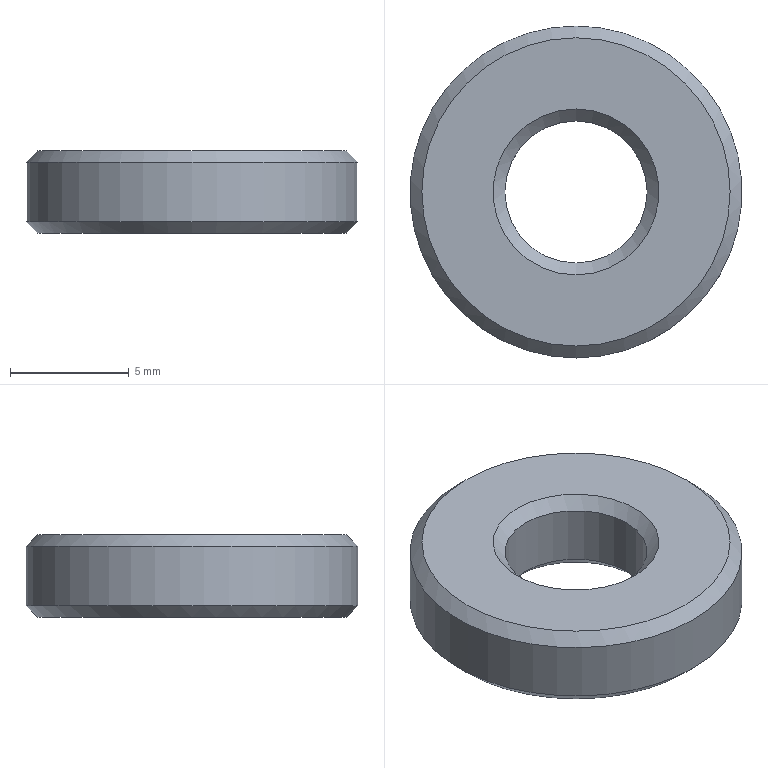Component | NX | STOPPER | 1 solid | 8 faces | box 14 x 14 x 3.5 mm | volume 424 mm3 | cone 4 | cylinder 2 | plane 2 | commonest cylinder face diameters 14 x1 6 x1
STEP:
#1=CARTESIAN_POINT('',(0.,0.,0.));
#2=DIRECTION('',(0.,0.,1.));
#3=DIRECTION('',(1.,0.,0.));
#4=AXIS2_PLACEMENT_3D('',#1,#2,#3);
#5=CARTESIAN_POINT('',(-8.293,7.,-172.611));
#6=VERTEX_POINT('',#5);
#7=CARTESIAN_POINT('',(-8.293,0.,-172.611));
#8=DIRECTION('',(0.,0.,-1.));
#9=DIRECTION('',(0.,1.,0.));
#10=AXIS2_PLACEMENT_3D('',#7,#8,#9);
#11=CIRCLE('',#10,7.);
#12=CARTESIAN_POINT('',(-8.293,0.,-175.611));
#13=DIRECTION('',(0.,0.,1.));
#14=DIRECTION('',(0.,1.,0.));
#15=AXIS2_PLACEMENT_3D('',#12,#13,#14);
#16=CYLINDRICAL_SURFACE('',#15,7.);
#17=CARTESIAN_POINT('',(6.283,3.));
#18=DIRECTION('',(-1.,0.));
#19=VECTOR('',#18,1.);
#20=LINE('',#17,#19);
#21=(GEOMETRIC_REPRESENTATION_CONTEXT(2)PARAMETRIC_REPRESENTATION_CONTEXT()REPRESENTATION_CONTEXT('',''));
#22=DEFINITIONAL_REPRESENTATION('',(#20),#21);
#23=PCURVE('',#16,#22);
#24=CARTESIAN_POINT('',(-8.293,0.,-172.111));
#25=DIRECTION('',(0.,0.,-1.));
#26=DIRECTION('',(0.,-1.,0.));
#27=AXIS2_PLACEMENT_3D('',#24,#25,#26);
#28=CONICAL_SURFACE('',#27,6.5,0.7854);
#29=CARTESIAN_POINT('',(3.142,0.5));
#30=DIRECTION('',(1.,0.));
#31=VECTOR('',#30,1.);
#32=LINE('',#29,#31);
#33=(GEOMETRIC_REPRESENTATION_CONTEXT(2)PARAMETRIC_REPRESENTATION_CONTEXT()REPRESENTATION_CONTEXT('',''));
#34=DEFINITIONAL_REPRESENTATION('',(#32),#33);
#35=PCURVE('',#28,#34);
#36=SURFACE_CURVE('',#11,(#23,#35),.PCURVE_S1.);
#37=EDGE_CURVE('',#6,#6,#36,.T.);
#38=ORIENTED_EDGE('',*,*,#37,.T.);
#39=CARTESIAN_POINT('',(-8.293,7.,-175.111));
#40=VERTEX_POINT('',#39);
#41=CARTESIAN_POINT('',(-8.293,7.,-175.111));
#42=CARTESIAN_POINT('',(-8.293,7.,-172.611));
#43=B_SPLINE_CURVE_WITH_KNOTS('',1,(#41,#42),.UNSPECIFIED.,.F.,.F.,(2,2),(0.5,3.),.PIECEWISE_BEZIER_KNOTS.);
#44=CARTESIAN_POINT('',(0.,0.));
#45=DIRECTION('',(0.,1.));
#46=VECTOR('',#45,1.);
#47=LINE('',#44,#46);
#48=(GEOMETRIC_REPRESENTATION_CONTEXT(2)PARAMETRIC_REPRESENTATION_CONTEXT()REPRESENTATION_CONTEXT('',''));
#49=DEFINITIONAL_REPRESENTATION('',(#47),#48);
#50=PCURVE('',#16,#49);
#51=CARTESIAN_POINT('',(6.283,0.));
#52=DIRECTION('',(0.,1.));
#53=VECTOR('',#52,1.);
#54=LINE('',#51,#53);
#55=(GEOMETRIC_REPRESENTATION_CONTEXT(2)PARAMETRIC_REPRESENTATION_CONTEXT()REPRESENTATION_CONTEXT('',''));
#56=DEFINITIONAL_REPRESENTATION('',(#54),#55);
#57=PCURVE('',#16,#56);
#58=SEAM_CURVE('',#43,(#50,#57),.PCURVE_S1.);
#59=EDGE_CURVE('',#40,#6,#58,.T.);
#60=ORIENTED_EDGE('',*,*,#59,.F.);
#61=CARTESIAN_POINT('',(-8.293,0.,-175.111));
#62=DIRECTION('',(0.,0.,1.));
#63=DIRECTION('',(0.,1.,0.));
#64=AXIS2_PLACEMENT_3D('',#61,#62,#63);
#65=CIRCLE('',#64,7.);
#66=CARTESIAN_POINT('',(0.,0.5));
#67=DIRECTION('',(1.,0.));
#68=VECTOR('',#67,1.);
#69=LINE('',#66,#68);
#70=(GEOMETRIC_REPRESENTATION_CONTEXT(2)PARAMETRIC_REPRESENTATION_CONTEXT()REPRESENTATION_CONTEXT('',''));
#71=DEFINITIONAL_REPRESENTATION('',(#69),#70);
#72=PCURVE('',#16,#71);
#73=CARTESIAN_POINT('',(-8.293,0.,-175.111));
#74=DIRECTION('',(0.,0.,1.));
#75=DIRECTION('',(0.,1.,0.));
#76=AXIS2_PLACEMENT_3D('',#73,#74,#75);
#77=CONICAL_SURFACE('',#76,7.,0.7854);
#78=CARTESIAN_POINT('',(0.,0.));
#79=DIRECTION('',(1.,0.));
#80=VECTOR('',#79,1.);
#81=LINE('',#78,#80);
#82=(GEOMETRIC_REPRESENTATION_CONTEXT(2)PARAMETRIC_REPRESENTATION_CONTEXT()REPRESENTATION_CONTEXT('',''));
#83=DEFINITIONAL_REPRESENTATION('',(#81),#82);
#84=PCURVE('',#77,#83);
#85=SURFACE_CURVE('',#65,(#72,#84),.PCURVE_S1.);
#86=EDGE_CURVE('',#40,#40,#85,.T.);
#87=ORIENTED_EDGE('',*,*,#86,.T.);
#88=ORIENTED_EDGE('',*,*,#59,.T.);
#89=EDGE_LOOP('',(#38,#60,#87,#88));
#90=FACE_BOUND('',#89,.T.);
#91=ADVANCED_FACE('',(#90),#16,.T.);
#92=CARTESIAN_POINT('',(-8.293,3.,-172.611));
#93=VERTEX_POINT('',#92);
#94=CARTESIAN_POINT('',(-8.293,0.,-172.611));
#95=DIRECTION('',(0.,0.,1.));
#96=DIRECTION('',(0.,1.,0.));
#97=AXIS2_PLACEMENT_3D('',#94,#95,#96);
#98=CIRCLE('',#97,3.);
#99=CARTESIAN_POINT('',(-8.293,0.,-175.611));
#100=DIRECTION('',(0.,0.,1.));
#101=DIRECTION('',(0.,1.,0.));
#102=AXIS2_PLACEMENT_3D('',#99,#100,#101);
#103=CYLINDRICAL_SURFACE('',#102,3.);
#104=CARTESIAN_POINT('',(0.,3.));
#105=DIRECTION('',(1.,0.));
#106=VECTOR('',#105,1.);
#107=LINE('',#104,#106);
#108=(GEOMETRIC_REPRESENTATION_CONTEXT(2)PARAMETRIC_REPRESENTATION_CONTEXT()REPRESENTATION_CONTEXT('',''));
#109=DEFINITIONAL_REPRESENTATION('',(#107),#108);
#110=PCURVE('',#103,#109);
#111=CARTESIAN_POINT('',(-8.293,0.,-172.611));
#112=DIRECTION('',(0.,0.,1.));
#113=DIRECTION('',(0.,1.,0.));
#114=AXIS2_PLACEMENT_3D('',#111,#112,#113);
#115=CONICAL_SURFACE('',#114,3.,0.7854);
#116=CARTESIAN_POINT('',(0.,0.));
#117=DIRECTION('',(1.,0.));
#118=VECTOR('',#117,1.);
#119=LINE('',#116,#118);
#120=(GEOMETRIC_REPRESENTATION_CONTEXT(2)PARAMETRIC_REPRESENTATION_CONTEXT()REPRESENTATION_CONTEXT('',''));
#121=DEFINITIONAL_REPRESENTATION('',(#119),#120);
#122=PCURVE('',#115,#121);
#123=SURFACE_CURVE('',#98,(#110,#122),.PCURVE_S1.);
#124=EDGE_CURVE('',#93,#93,#123,.T.);
#125=ORIENTED_EDGE('',*,*,#124,.F.);
#126=CARTESIAN_POINT('',(-8.293,3.,-175.111));
#127=VERTEX_POINT('',#126);
#128=CARTESIAN_POINT('',(-8.293,3.,-175.111));
#129=CARTESIAN_POINT('',(-8.293,3.,-172.611));
#130=B_SPLINE_CURVE_WITH_KNOTS('',1,(#128,#129),.UNSPECIFIED.,.F.,.F.,(2,2),(0.5,3.),.PIECEWISE_BEZIER_KNOTS.);
#131=CARTESIAN_POINT('',(0.,0.));
#132=DIRECTION('',(0.,1.));
#133=VECTOR('',#132,1.);
#134=LINE('',#131,#133);
#135=(GEOMETRIC_REPRESENTATION_CONTEXT(2)PARAMETRIC_REPRESENTATION_CONTEXT()REPRESENTATION_CONTEXT('',''));
#136=DEFINITIONAL_REPRESENTATION('',(#134),#135);
#137=PCURVE('',#103,#136);
#138=CARTESIAN_POINT('',(6.283,0.));
#139=DIRECTION('',(0.,1.));
#140=VECTOR('',#139,1.);
#141=LINE('',#138,#140);
#142=(GEOMETRIC_REPRESENTATION_CONTEXT(2)PARAMETRIC_REPRESENTATION_CONTEXT()REPRESENTATION_CONTEXT('',''));
#143=DEFINITIONAL_REPRESENTATION('',(#141),#142);
#144=PCURVE('',#103,#143);
#145=SEAM_CURVE('',#130,(#137,#144),.PCURVE_S1.);
#146=EDGE_CURVE('',#127,#93,#145,.T.);
#147=ORIENTED_EDGE('',*,*,#146,.F.);
#148=CARTESIAN_POINT('',(-8.293,0.,-175.111));
#149=DIRECTION('',(0.,0.,-1.));
#150=DIRECTION('',(0.,1.,0.));
#151=AXIS2_PLACEMENT_3D('',#148,#149,#150);
#152=CIRCLE('',#151,3.);
#153=CARTESIAN_POINT('',(6.283,0.5));
#154=DIRECTION('',(-1.,0.));
#155=VECTOR('',#154,1.);
#156=LINE('',#153,#155);
#157=(GEOMETRIC_REPRESENTATION_CONTEXT(2)PARAMETRIC_REPRESENTATION_CONTEXT()REPRESENTATION_CONTEXT('',''));
#158=DEFINITIONAL_REPRESENTATION('',(#156),#157);
#159=PCURVE('',#103,#158);
#160=CARTESIAN_POINT('',(-8.293,0.,-175.611));
#161=DIRECTION('',(0.,0.,-1.));
#162=DIRECTION('',(0.,-1.,0.));
#163=AXIS2_PLACEMENT_3D('',#160,#161,#162);
#164=CONICAL_SURFACE('',#163,3.5,0.7854);
#165=CARTESIAN_POINT('',(3.142,-0.5));
#166=DIRECTION('',(1.,0.));
#167=VECTOR('',#166,1.);
#168=LINE('',#165,#167);
#169=(GEOMETRIC_REPRESENTATION_CONTEXT(2)PARAMETRIC_REPRESENTATION_CONTEXT()REPRESENTATION_CONTEXT('',''));
#170=DEFINITIONAL_REPRESENTATION('',(#168),#169);
#171=PCURVE('',#164,#170);
#172=SURFACE_CURVE('',#152,(#159,#171),.PCURVE_S1.);
#173=EDGE_CURVE('',#127,#127,#172,.T.);
#174=ORIENTED_EDGE('',*,*,#173,.F.);
#175=ORIENTED_EDGE('',*,*,#146,.T.);
#176=EDGE_LOOP('',(#125,#147,#174,#175));
#177=FACE_BOUND('',#176,.F.);
#178=ADVANCED_FACE('',(#177),#103,.F.);
#179=CARTESIAN_POINT('',(-8.293,6.5,-175.611));
#180=VERTEX_POINT('',#179);
#181=CARTESIAN_POINT('',(-8.293,0.,-175.611));
#182=DIRECTION('',(0.,0.,-1.));
#183=DIRECTION('',(0.,1.,0.));
#184=AXIS2_PLACEMENT_3D('',#181,#182,#183);
#185=CIRCLE('',#184,6.5);
#186=CARTESIAN_POINT('',(-8.293,0.,-175.611));
#187=DIRECTION('',(0.,0.,1.));
#188=DIRECTION('',(0.,1.,0.));
#189=AXIS2_PLACEMENT_3D('',#186,#187,#188);
#190=PLANE('',#189);
#191=CARTESIAN_POINT('',(6.5,0.));
#192=CARTESIAN_POINT('',(6.5,-11.258));
#193=CARTESIAN_POINT('',(-3.25,-5.629));
#194=CARTESIAN_POINT('',(-13.,-0.));
#195=CARTESIAN_POINT('',(-3.25,5.629));
#196=CARTESIAN_POINT('',(6.5,11.258));
#197=CARTESIAN_POINT('',(6.5,0.));
#198=(BOUNDED_CURVE()B_SPLINE_CURVE(2,(#191,#192,#193,#194,#195,#196,#197),.UNSPECIFIED.,.T.,.F.)B_SPLINE_CURVE_WITH_KNOTS((1,2,2,2,2,1),(-2.094,0.,2.094,4.189,6.283,8.378),.UNSPECIFIED.)CURVE()GEOMETRIC_REPRESENTATION_ITEM()RATIONAL_B_SPLINE_CURVE((1.,0.5,1.,0.5,1.,0.5,1.))REPRESENTATION_ITEM(''));
#199=(GEOMETRIC_REPRESENTATION_CONTEXT(2)PARAMETRIC_REPRESENTATION_CONTEXT()REPRESENTATION_CONTEXT('',''));
#200=DEFINITIONAL_REPRESENTATION('',(#198),#199);
#201=PCURVE('',#190,#200);
#202=CARTESIAN_POINT('',(6.283,-0.5));
#203=DIRECTION('',(-1.,0.));
#204=VECTOR('',#203,1.);
#205=LINE('',#202,#204);
#206=(GEOMETRIC_REPRESENTATION_CONTEXT(2)PARAMETRIC_REPRESENTATION_CONTEXT()REPRESENTATION_CONTEXT('',''));
#207=DEFINITIONAL_REPRESENTATION('',(#205),#206);
#208=PCURVE('',#77,#207);
#209=SURFACE_CURVE('',#185,(#201,#208),.PCURVE_S1.);
#210=EDGE_CURVE('',#180,#180,#209,.T.);
#211=ORIENTED_EDGE('',*,*,#210,.T.);
#212=EDGE_LOOP('',(#211));
#213=FACE_BOUND('',#212,.T.);
#214=CARTESIAN_POINT('',(-8.293,3.5,-175.611));
#215=VERTEX_POINT('',#214);
#216=CARTESIAN_POINT('',(-8.293,0.,-175.611));
#217=DIRECTION('',(0.,0.,1.));
#218=DIRECTION('',(0.,1.,0.));
#219=AXIS2_PLACEMENT_3D('',#216,#217,#218);
#220=CIRCLE('',#219,3.5);
#221=CARTESIAN_POINT('',(0.,0.));
#222=DIRECTION('',(1.,0.));
#223=AXIS2_PLACEMENT_2D('',#221,#222);
#224=CIRCLE('',#223,3.5);
#225=(GEOMETRIC_REPRESENTATION_CONTEXT(2)PARAMETRIC_REPRESENTATION_CONTEXT()REPRESENTATION_CONTEXT('',''));
#226=DEFINITIONAL_REPRESENTATION('',(#224),#225);
#227=PCURVE('',#190,#226);
#228=CARTESIAN_POINT('',(9.425,0.));
#229=DIRECTION('',(-1.,0.));
#230=VECTOR('',#229,1.);
#231=LINE('',#228,#230);
#232=(GEOMETRIC_REPRESENTATION_CONTEXT(2)PARAMETRIC_REPRESENTATION_CONTEXT()REPRESENTATION_CONTEXT('',''));
#233=DEFINITIONAL_REPRESENTATION('',(#231),#232);
#234=PCURVE('',#164,#233);
#235=SURFACE_CURVE('',#220,(#227,#234),.PCURVE_S1.);
#236=EDGE_CURVE('',#215,#215,#235,.T.);
#237=ORIENTED_EDGE('',*,*,#236,.T.);
#238=EDGE_LOOP('',(#237));
#239=FACE_BOUND('',#238,.T.);
#240=ADVANCED_FACE('',(#213,#239),#190,.F.);
#241=CARTESIAN_POINT('',(-8.293,3.5,-172.111));
#242=VERTEX_POINT('',#241);
#243=CARTESIAN_POINT('',(-8.293,0.,-172.111));
#244=DIRECTION('',(0.,0.,-1.));
#245=DIRECTION('',(0.,1.,0.));
#246=AXIS2_PLACEMENT_3D('',#243,#244,#245);
#247=CIRCLE('',#246,3.5);
#248=CARTESIAN_POINT('',(-8.293,0.,-172.111));
#249=DIRECTION('',(0.,0.,1.));
#250=DIRECTION('',(0.,1.,0.));
#251=AXIS2_PLACEMENT_3D('',#248,#249,#250);
#252=PLANE('',#251);
#253=CARTESIAN_POINT('',(3.5,0.));
#254=CARTESIAN_POINT('',(3.5,-6.062));
#255=CARTESIAN_POINT('',(-1.75,-3.031));
#256=CARTESIAN_POINT('',(-7.,-0.));
#257=CARTESIAN_POINT('',(-1.75,3.031));
#258=CARTESIAN_POINT('',(3.5,6.062));
#259=CARTESIAN_POINT('',(3.5,0.));
#260=(BOUNDED_CURVE()B_SPLINE_CURVE(2,(#253,#254,#255,#256,#257,#258,#259),.UNSPECIFIED.,.T.,.F.)B_SPLINE_CURVE_WITH_KNOTS((1,2,2,2,2,1),(-2.094,0.,2.094,4.189,6.283,8.378),.UNSPECIFIED.)CURVE()GEOMETRIC_REPRESENTATION_ITEM()RATIONAL_B_SPLINE_CURVE((1.,0.5,1.,0.5,1.,0.5,1.))REPRESENTATION_ITEM(''));
#261=(GEOMETRIC_REPRESENTATION_CONTEXT(2)PARAMETRIC_REPRESENTATION_CONTEXT()REPRESENTATION_CONTEXT('',''));
#262=DEFINITIONAL_REPRESENTATION('',(#260),#261);
#263=PCURVE('',#252,#262);
#264=CARTESIAN_POINT('',(6.283,0.5));
#265=DIRECTION('',(-1.,0.));
#266=VECTOR('',#265,1.);
#267=LINE('',#264,#266);
#268=(GEOMETRIC_REPRESENTATION_CONTEXT(2)PARAMETRIC_REPRESENTATION_CONTEXT()REPRESENTATION_CONTEXT('',''));
#269=DEFINITIONAL_REPRESENTATION('',(#267),#268);
#270=PCURVE('',#115,#269);
#271=SURFACE_CURVE('',#247,(#263,#270),.PCURVE_S1.);
#272=EDGE_CURVE('',#242,#242,#271,.T.);
#273=ORIENTED_EDGE('',*,*,#272,.T.);
#274=EDGE_LOOP('',(#273));
#275=FACE_BOUND('',#274,.T.);
#276=CARTESIAN_POINT('',(-8.293,6.5,-172.111));
#277=VERTEX_POINT('',#276);
#278=CARTESIAN_POINT('',(-8.293,0.,-172.111));
#279=DIRECTION('',(0.,0.,1.));
#280=DIRECTION('',(0.,1.,0.));
#281=AXIS2_PLACEMENT_3D('',#278,#279,#280);
#282=CIRCLE('',#281,6.5);
#283=CARTESIAN_POINT('',(0.,0.));
#284=DIRECTION('',(1.,0.));
#285=AXIS2_PLACEMENT_2D('',#283,#284);
#286=CIRCLE('',#285,6.5);
#287=(GEOMETRIC_REPRESENTATION_CONTEXT(2)PARAMETRIC_REPRESENTATION_CONTEXT()REPRESENTATION_CONTEXT('',''));
#288=DEFINITIONAL_REPRESENTATION('',(#286),#287);
#289=PCURVE('',#252,#288);
#290=CARTESIAN_POINT('',(9.425,0.));
#291=DIRECTION('',(-1.,0.));
#292=VECTOR('',#291,1.);
#293=LINE('',#290,#292);
#294=(GEOMETRIC_REPRESENTATION_CONTEXT(2)PARAMETRIC_REPRESENTATION_CONTEXT()REPRESENTATION_CONTEXT('',''));
#295=DEFINITIONAL_REPRESENTATION('',(#293),#294);
#296=PCURVE('',#28,#295);
#297=SURFACE_CURVE('',#282,(#289,#296),.PCURVE_S1.);
#298=EDGE_CURVE('',#277,#277,#297,.T.);
#299=ORIENTED_EDGE('',*,*,#298,.T.);
#300=EDGE_LOOP('',(#299));
#301=FACE_BOUND('',#300,.T.);
#302=ADVANCED_FACE('',(#275,#301),#252,.T.);
#303=ORIENTED_EDGE('',*,*,#272,.T.);
#304=CARTESIAN_POINT('',(-8.293,3.,-172.611));
#305=CARTESIAN_POINT('',(-8.293,3.5,-172.111));
#306=B_SPLINE_CURVE_WITH_KNOTS('',1,(#304,#305),.UNSPECIFIED.,.F.,.F.,(2,2),(0.,0.7071),.PIECEWISE_BEZIER_KNOTS.);
#307=CARTESIAN_POINT('',(0.,0.));
#308=DIRECTION('',(0.,1.));
#309=VECTOR('',#308,1.);
#310=LINE('',#307,#309);
#311=(GEOMETRIC_REPRESENTATION_CONTEXT(2)PARAMETRIC_REPRESENTATION_CONTEXT()REPRESENTATION_CONTEXT('',''));
#312=DEFINITIONAL_REPRESENTATION('',(#310),#311);
#313=PCURVE('',#115,#312);
#314=CARTESIAN_POINT('',(6.283,0.));
#315=DIRECTION('',(0.,1.));
#316=VECTOR('',#315,1.);
#317=LINE('',#314,#316);
#318=(GEOMETRIC_REPRESENTATION_CONTEXT(2)PARAMETRIC_REPRESENTATION_CONTEXT()REPRESENTATION_CONTEXT('',''));
#319=DEFINITIONAL_REPRESENTATION('',(#317),#318);
#320=PCURVE('',#115,#319);
#321=SEAM_CURVE('',#306,(#313,#320),.PCURVE_S1.);
#322=EDGE_CURVE('',#93,#242,#321,.T.);
#323=ORIENTED_EDGE('',*,*,#322,.F.);
#324=ORIENTED_EDGE('',*,*,#124,.T.);
#325=ORIENTED_EDGE('',*,*,#322,.T.);
#326=EDGE_LOOP('',(#303,#323,#324,#325));
#327=FACE_BOUND('',#326,.F.);
#328=ADVANCED_FACE('',(#327),#115,.F.);
#329=ORIENTED_EDGE('',*,*,#37,.F.);
#330=CARTESIAN_POINT('',(-8.293,6.5,-172.111));
#331=CARTESIAN_POINT('',(-8.293,7.,-172.611));
#332=B_SPLINE_CURVE_WITH_KNOTS('',1,(#330,#331),.UNSPECIFIED.,.F.,.F.,(2,2),(0.,0.7071),.PIECEWISE_BEZIER_KNOTS.);
#333=CARTESIAN_POINT('',(3.142,0.));
#334=DIRECTION('',(0.,1.));
#335=VECTOR('',#334,1.);
#336=LINE('',#333,#335);
#337=(GEOMETRIC_REPRESENTATION_CONTEXT(2)PARAMETRIC_REPRESENTATION_CONTEXT()REPRESENTATION_CONTEXT('',''));
#338=DEFINITIONAL_REPRESENTATION('',(#336),#337);
#339=PCURVE('',#28,#338);
#340=CARTESIAN_POINT('',(9.425,0.));
#341=DIRECTION('',(0.,1.));
#342=VECTOR('',#341,1.);
#343=LINE('',#340,#342);
#344=(GEOMETRIC_REPRESENTATION_CONTEXT(2)PARAMETRIC_REPRESENTATION_CONTEXT()REPRESENTATION_CONTEXT('',''));
#345=DEFINITIONAL_REPRESENTATION('',(#343),#344);
#346=PCURVE('',#28,#345);
#347=SEAM_CURVE('',#332,(#339,#346),.PCURVE_S1.);
#348=EDGE_CURVE('',#277,#6,#347,.T.);
#349=ORIENTED_EDGE('',*,*,#348,.F.);
#350=ORIENTED_EDGE('',*,*,#298,.F.);
#351=ORIENTED_EDGE('',*,*,#348,.T.);
#352=EDGE_LOOP('',(#329,#349,#350,#351));
#353=FACE_BOUND('',#352,.T.);
#354=ADVANCED_FACE('',(#353),#28,.T.);
#355=ORIENTED_EDGE('',*,*,#210,.F.);
#356=CARTESIAN_POINT('',(-8.293,6.5,-175.611));
#357=CARTESIAN_POINT('',(-8.293,7.,-175.111));
#358=B_SPLINE_CURVE_WITH_KNOTS('',1,(#356,#357),.UNSPECIFIED.,.F.,.F.,(2,2),(-0.7071,0.),.PIECEWISE_BEZIER_KNOTS.);
#359=CARTESIAN_POINT('',(6.283,0.));
#360=DIRECTION('',(0.,1.));
#361=VECTOR('',#360,1.);
#362=LINE('',#359,#361);
#363=(GEOMETRIC_REPRESENTATION_CONTEXT(2)PARAMETRIC_REPRESENTATION_CONTEXT()REPRESENTATION_CONTEXT('',''));
#364=DEFINITIONAL_REPRESENTATION('',(#362),#363);
#365=PCURVE('',#77,#364);
#366=CARTESIAN_POINT('',(0.,0.));
#367=DIRECTION('',(0.,1.));
#368=VECTOR('',#367,1.);
#369=LINE('',#366,#368);
#370=(GEOMETRIC_REPRESENTATION_CONTEXT(2)PARAMETRIC_REPRESENTATION_CONTEXT()REPRESENTATION_CONTEXT('',''));
#371=DEFINITIONAL_REPRESENTATION('',(#369),#370);
#372=PCURVE('',#77,#371);
#373=SEAM_CURVE('',#358,(#365,#372),.PCURVE_S1.);
#374=EDGE_CURVE('',#180,#40,#373,.T.);
#375=ORIENTED_EDGE('',*,*,#374,.T.);
#376=ORIENTED_EDGE('',*,*,#86,.F.);
#377=ORIENTED_EDGE('',*,*,#374,.F.);
#378=EDGE_LOOP('',(#355,#375,#376,#377));
#379=FACE_BOUND('',#378,.T.);
#380=ADVANCED_FACE('',(#379),#77,.T.);
#381=ORIENTED_EDGE('',*,*,#173,.T.);
#382=CARTESIAN_POINT('',(-8.293,3.,-175.111));
#383=CARTESIAN_POINT('',(-8.293,3.5,-175.611));
#384=B_SPLINE_CURVE_WITH_KNOTS('',1,(#382,#383),.UNSPECIFIED.,.F.,.F.,(2,2),(-0.7071,0.),.PIECEWISE_BEZIER_KNOTS.);
#385=CARTESIAN_POINT('',(9.425,0.));
#386=DIRECTION('',(0.,1.));
#387=VECTOR('',#386,1.);
#388=LINE('',#385,#387);
#389=(GEOMETRIC_REPRESENTATION_CONTEXT(2)PARAMETRIC_REPRESENTATION_CONTEXT()REPRESENTATION_CONTEXT('',''));
#390=DEFINITIONAL_REPRESENTATION('',(#388),#389);
#391=PCURVE('',#164,#390);
#392=CARTESIAN_POINT('',(3.142,0.));
#393=DIRECTION('',(0.,1.));
#394=VECTOR('',#393,1.);
#395=LINE('',#392,#394);
#396=(GEOMETRIC_REPRESENTATION_CONTEXT(2)PARAMETRIC_REPRESENTATION_CONTEXT()REPRESENTATION_CONTEXT('',''));
#397=DEFINITIONAL_REPRESENTATION('',(#395),#396);
#398=PCURVE('',#164,#397);
#399=SEAM_CURVE('',#384,(#391,#398),.PCURVE_S1.);
#400=EDGE_CURVE('',#127,#215,#399,.T.);
#401=ORIENTED_EDGE('',*,*,#400,.T.);
#402=ORIENTED_EDGE('',*,*,#236,.T.);
#403=ORIENTED_EDGE('',*,*,#400,.F.);
#404=EDGE_LOOP('',(#381,#401,#402,#403));
#405=FACE_BOUND('',#404,.F.);
#406=ADVANCED_FACE('',(#405),#164,.F.);
#407=CLOSED_SHELL('',(#91,#178,#240,#302,#328,#354,#380,#406));
#408=MANIFOLD_SOLID_BREP('',#407);
#409=(LENGTH_UNIT()NAMED_UNIT(*)SI_UNIT(.MILLI.,.METRE.));
#410=UNCERTAINTY_MEASURE_WITH_UNIT(LENGTH_MEASURE(0.00001),#409,'','');
#411=(NAMED_UNIT(*)PLANE_ANGLE_UNIT()SI_UNIT($,.RADIAN.));
#412=(NAMED_UNIT(*)SI_UNIT($,.STERADIAN.)SOLID_ANGLE_UNIT());
#413=(GEOMETRIC_REPRESENTATION_CONTEXT(3)GLOBAL_UNCERTAINTY_ASSIGNED_CONTEXT((#410))GLOBAL_UNIT_ASSIGNED_CONTEXT((#409,#411,#412))REPRESENTATION_CONTEXT('',''));
#414=ADVANCED_BREP_SHAPE_REPRESENTATION('',(#4,#408),#413);